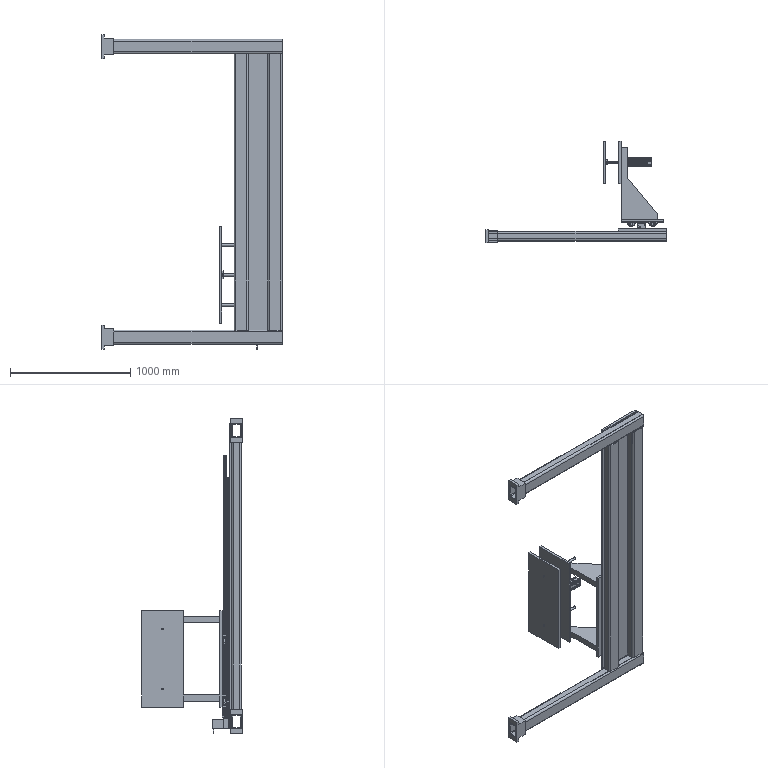Assembly | SolidWorks | mm | 26 component files | 26 solids | 1495 faces | box 1500 x 840 x 2621.5 mm | volume 76964541 mm3 | plane 802 | cylinder 635 | cone 42 | spline 16 | commonest cylinder face diameters 11 x160 7 x154 8 x48 5.5 x42 4.6 x24 4.26 x18 32 x16 16 x16
Bill of materials:
CQ2A50-200DCZ(0_0_0)1 | 1 |  | Long prismatic profile with a square-like cross-section. Each of the four corners has a rounded lobe with a round through-hole along the length. There are long grooves/slots on the faces and a small rectangular tab sticking out from one side at one end.
CQ2A50-200DCZ(0_0_0)2 | 1 |  | Headed pin: a long cylindrical shank with a thin, flat, round head at one end and a small step or chamfer at the other end.
HG_BLOCK_HGWHC_ANY | 4 |  | Block with a wide top flange and a narrower tapered lower body. A central open channel runs lengthwise through the underside. The flange has four through-holes and the side faces have curved pockets.
HG_RAIL0_R_ANY_1 | 2 |  | Very long, slender prismatic bar with a constant, complex cross-section. Concave semicircular notches are cut into the upper side edges, the lower part is chamfered, and there are two shallow notches in the bottom face.
LEFB32T-1800(0_0_0)1 | 1 |  | Long, slender L-shaped member: a straight bar with a short foot bent at one end. One view shows a broad rectangular face with rounded side edges, two small bosses and a small hole near one corner.
LEFB32T-1800(0_0_0)2 | 1 |  | Thin rectangular plate or cap with slightly tapered, rounded ends. Two longitudinal grooves run along its main face, and the edges are stepped.
ST60-02 | 2 |  | Straight rectangular hollow tube with rounded outer and inner corners and square-cut ends.
ST60-03 | 2 |  | Short rectangular hollow box section attached to a flat square plate at one end. The plate extends beyond the tube walls.
ST60-04 | 2 |  | Long rectangular hollow tube with rounded corners, uniform wall thickness and square-cut ends.
ST60-05 | 1 |  | Thin, flat, long rectangular strip of uniform thickness with no visible holes or cutouts.
ST60-06 | 1 |  | Thin, flat rectangular plate of uniform thickness with no visible holes, cutouts or edge features.
ST60-07 | 2 |  | Flat plate of uniform thickness shaped like a gusset: a narrow straight strip that widens along an angled edge into a broad, roughly trapezoidal end.
ST60-08 | 1 |  | Thin flat rectangular plate with three through holes in a line along the long centerline: a larger hole in the middle and a smaller hole near each end.
ST60-10 | 1 |  | Thin flat rectangular plate, similar in outline to a plain panel, with two very small holes on the long centerline, one near each end.
ST60-11 | 2 |  | Plain solid round rod or cylinder, long relative to its diameter, with flat ends.
ST60-12 | 1 |  | Thick rectangular block with a U-shaped slot open on one long side at mid-length and a round through hole on each side of the slot. A small step is visible near the slot opening.
ST60-13 | 1 |  | Hollow round tube with a short, larger-diameter flange at one end and a through bore along its axis, like a flanged sleeve or bushing.
Mates:
1. coincident | ST60-02-1 face at (-847.007, 19.454, 44) dir (-1, 0, 0) | ST60-03-1 face at (-847.007, 45.454, 100) dir (-1, 0, 0)
2. coincident | ST60-02-1 face at (652.993, -44.546, -44) dir (0, -1, 0) | ST60-03-1 face at (-847.007, -44.546, -60) dir (0, 1, 0)
3. coincident | ST60-02-1 face at (652.993, 19.454, 60) dir (0, 0, 1) | ST60-03-1 face at (-847.007, -44.546, 60) dir (0, 0, -1)
4. coincident | ST60-02-3 face at (652.993, 35.454, -2376) dir (0, 1, 0) | ST60-03-2 face at (-847.007, 35.454, -2480) dir (0, -1, 0)
5. coincident | ST60-02-3 face at (652.993, 19.454, -2360) dir (0, 0, 1) | ST60-03-2 face at (-847.007, -44.546, -2360) dir (0, 0, -1)
6. coincident | ST60-02-3 face at (-847.007, 19.454, -2376) dir (-1, 0, 0) | ST60-03-2 face at (-847.007, 45.454, -2320) dir (-1, 0, 0)
7. coincident | ST60-02-1 face at (652.993, -28.546, -60) dir (0, 0, -1) | ST60-04-1 face at (548.993, 19.454, -60) dir (0, 0, 1)
8. coincident | ST60-02-1 face at (652.993, -44.546, -44) dir (0, -1, 0) | ST60-04-1 face at (636.993, -44.546, -60) dir (0, -1, 0)
9. coincident | ST60-02-1 face at (652.993, 19.454, 44) dir (1, 0, 0) | ST60-04-1 face at (652.993, -28.546, -60) dir (1, 0, 0)
10. coincident | ST60-02-1 face at (652.993, -44.546, -44) dir (0, -1, 0) | ST60-02-3 face at (652.993, -44.546, -2464) dir (0, -1, 0)
11. coincident | ST60-02-1 face at (652.993, 19.454, 44) dir (1, 0, 0) | ST60-02-3 face at (652.993, 19.454, -2376) dir (1, 0, 0)
12. coincident | ST60-02-3 face at (652.993, 19.454, -2360) dir (0, 0, 1) | ST60-04-1 face at (548.993, 19.454, -2360) dir (0, 0, -1)
13. coincident | ST60-02-1 face at (652.993, -44.546, -44) dir (0, -1, 0) | ST60-04-2 face at (356.993, -44.546, -60) dir (0, -1, 0)
14. coincident | ST60-02-1 face at (652.993, -28.546, -60) dir (0, 0, -1) | ST60-04-2 face at (268.993, 19.454, -60) dir (0, 0, 1)
15. coincident | ST60-02-3 face at (652.993, -28.546, -2480) dir (0, 0, -1) | ST60-05-1 face at (252.993, 35.454, -2480) dir (0, 0, -1)
16. coincident | ST60-04-1 face at (652.993, -28.546, -60) dir (1, 0, 0) | ST60-05-1 face at (652.993, 35.454, -2480) dir (1, 0, 0)
17. coincident | ST60-02-3 face at (652.993, 35.454, -2376) dir (0, 1, 0) | ST60-05-1 face at (969.968, 35.454, -955.511) dir (0, -1, 0)
18. parallel | HG_RAIL0_R_ANY_1-1 face at (351.493, 101.454, -2378.228) dir (0, 1, 0) | HG_BLOCK_HGWHC_ANY-2 face at (357.193, 115.254, -2189.672) dir (0, 1, 0)
19. concentric | HG_RAIL0_R_ANY_1-1 face at (373.988, 100.949, -2346.4) dir (0, 0, 1) r 2.3 | HG_BLOCK_HGWHC_ANY-2 face at (373.988, 100.949, -2194.795) dir (0, 0, -1) r 2.3
20. coincident | HG_BLOCK_HGWHC_ANY-1 face at (380.493, 114.954, -1710.8) dir (0, 1, 0) | HG_BLOCK_HGWHC_ANY-2 face at (380.493, 114.954, -2210.8) dir (0, 1, 0)
21. coincident | HG_BLOCK_HGWHC_ANY-1 face at (397.993, 115.454, -1634.444) dir (1, 0, 0) | HG_BLOCK_HGWHC_ANY-2 face at (397.993, 115.454, -2134.444) dir (1, 0, 0)
22. distance | HG_BLOCK_HGWHC_ANY-2 face at (351.493, 79.454, -2301.4) dir (0, 0, -1) | HG_RAIL0_R_ANY_1-1 face at (351.999, 91.91, -2351.4) dir (0, 0, -1)
23. distance | HG_BLOCK_HGWHC_ANY-1 face at (351.493, 79.454, -1801.4) dir (0, 0, -1) | HG_BLOCK_HGWHC_ANY-2 face at (351.493, 79.454, -2301.4) dir (0, 0, -1)
24. distance | HG_RAIL0_R_ANY_1-1 face at (351.999, 91.91, -2351.4) dir (0, 0, -1) | LEFB32T-1800(0_0_0)-1/LEFB32T-1800(0_0_0)1-1 face at (478.951, 100.254, -2401.4) dir (0, 0, 1)
25. coincident | LEFB32T-1800(0_0_0)-1/LEFB32T-1800(0_0_0)2-1 face at (447.151, 115.454, -2390.4) dir (0, 1, 0) | ST60-06-1 face at (994.968, 115.454, -776.911) dir (0, -1, 0)
26. coincident | HG_BLOCK_HGWHC_ANY-2 face at (327.993, 115.454, -2134.444) dir (0, 1, 0) | ST60-06-1 face at (994.968, 115.454, -776.911) dir (0, -1, 0)
27. distance | HG_BLOCK_HGWHC_ANY-2 face at (327.993, 115.454, -2134.444) dir (-1, 0, 0) | ST60-06-1 face at (277.993, 115.454, -2301.4) dir (-1, 0, 0)
28. coincident | HG_BLOCK_HGWHC_ANY-1 face at (327.993, 115.454, -1634.444) dir (-1, 0, 0) | HG_BLOCK_HGWHC_ANY-2 face at (327.993, 115.454, -2134.444) dir (-1, 0, 0)
29. coincident | HG_BLOCK_HGWHC_ANY-3 face at (507.993, 115.454, -1634.444) dir (0, 1, 0) | HG_BLOCK_HGWHC_ANY-4 face at (507.993, 115.454, -2134.444) dir (0, 1, 0)
30. coincident | HG_BLOCK_HGWHC_ANY-3 face at (507.993, 115.454, -1634.444) dir (-1, 0, 0) | HG_BLOCK_HGWHC_ANY-4 face at (507.993, 115.454, -2134.444) dir (-1, 0, 0)
31. concentric | HG_RAIL0_R_ANY_1-2 face at (531.999, 100.949, -2346.4) dir (0, 0, 1) r 2.3 | HG_BLOCK_HGWHC_ANY-3 face at (531.999, 100.949, -1694.795) dir (0, 0, -1) r 2.3
32. parallel | HG_RAIL0_R_ANY_1-2 face at (531.493, 101.454, -2378.228) dir (0, 1, 0) | HG_BLOCK_HGWHC_ANY-3 face at (507.993, 115.454, -1634.444) dir (0, 1, 0)
33. coincident | ST60-06-1 face at (994.968, 115.454, -776.911) dir (0, -1, 0) | HG_BLOCK_HGWHC_ANY-4 face at (507.993, 115.454, -2134.444) dir (0, 1, 0)
34. coincident | HG_RAIL0_R_ANY_1-1 face at (373.988, 91.91, -211.4) dir (0, 0, 1) | HG_RAIL0_R_ANY_1-2 face at (553.988, 91.91, -211.4) dir (0, 0, 1)
35. coincident | HG_BLOCK_HGWHC_ANY-1 face at (374.493, 79.454, -1698.8) dir (0, 0, 1) | HG_BLOCK_HGWHC_ANY-3 face at (554.493, 79.454, -1698.8) dir (0, 0, 1)
36. coincident | HG_BLOCK_HGWHC_ANY-2 face at (351.493, 79.454, -2301.4) dir (0, 0, -1) | HG_BLOCK_HGWHC_ANY-4 face at (531.493, 79.454, -2301.4) dir (0, 0, -1)
37. distance | HG_BLOCK_HGWHC_ANY-4 face at (577.993, 115.454, -2134.444) dir (1, 0, 0) | ST60-06-1 face at (627.993, 115.454, -2301.4) dir (1, 0, 0)
38. coincident | ST60-05-1 face at (969.968, 55.454, -955.511) dir (0, 1, 0) | LEFB32T-1800(0_0_0)-1/LEFB32T-1800(0_0_0)1-1 face at (480.151, 55.454, -2393.4) dir (0, -1, 0)
39. coincident | ST60-06-1 face at (994.968, 135.454, -776.911) dir (0, 1, 0) | ST60-07-1 face at (577.993, 135.454, -2251.4) dir (0, -1, 0)
40. parallel | ST60-06-1 face at (627.993, 115.454, -2301.4) dir (1, 0, 0) | ST60-07-1 face at (277.993, 135.454, -2251.4) dir (-1, 0, 0)
41. coincident | ST60-06-1 face at (277.993, 115.454, -2301.4) dir (-1, 0, 0) | ST60-07-1 face at (277.993, 135.454, -2251.4) dir (-1, 0, 0)
42. distance | ST60-07-1 face at (277.993, 135.454, -2251.4) dir (0, 0, -1) | ST60-06-1 face at (277.993, 115.454, -2301.4) dir (0, 0, -1)
43. coincident | ST60-06-1 face at (994.968, 135.454, -776.911) dir (0, 1, 0) | ST60-07-2 face at (577.993, 135.454, -1601.4) dir (0, -1, 0)
44. distance | ST60-07-2 face at (277.993, 135.454, -1551.4) dir (0, 0, 1) | ST60-06-1 face at (277.993, 115.454, -1501.4) dir (0, 0, 1)
45. coincident | ST60-07-1 face at (327.993, 735.454, -2251.4) dir (1, 0, 0) | ST60-07-2 face at (327.993, 735.454, -1601.4) dir (1, 0, 0)
46. coincident | ST60-07-1 face at (277.993, 135.454, -2251.4) dir (-1, 0, 0) | ST60-08-1 face at (277.993, 68.479, -776.911) dir (1, 0, 0)
47. width | ST60-08-1 face at (257.993, 785.454, -2301.4) dir (0, 0, -1) | ST60-08-1 face at (257.993, 785.454, -1501.4) dir (0, 0, 1) | ST60-07-2 face at (277.993, 135.454, -1551.4) dir (0, 0, 1) | ST60-07-1 face at (277.993, 135.454, -2251.4) dir (0, 0, -1)
48. coincident | ST60-07-2 face at (277.993, 135.454, -1601.4) dir (-1, 0, 0) | ST60-08-1 face at (277.993, 68.479, -776.911) dir (1, 0, 0)
49. distance | ST60-06-1 face at (277.993, 115.454, -2301.4) dir (0, 0, -1) | LEFB32T-1800(0_0_0)-1/LEFB32T-1800(0_0_0)1-1 face at (478.951, 100.254, -2401.4) dir (0, 0, 1)
50. distance | ST60-07-1 face at (277.993, 735.454, -2251.4) dir (0, 1, 0) | ST60-08-1 face at (257.993, 785.454, -2301.4) dir (0, 1, 0)
51. width | ST60-06-1 face at (627.993, 115.454, -2301.4) dir (1, 0, 0) | ST60-06-1 face at (277.993, 115.454, -2301.4) dir (-1, 0, 0) | ST60-05-1 face at (252.993, 35.454, -2480) dir (-1, 0, 0) | ST60-05-1 face at (652.993, 35.454, -2480) dir (1, 0, 0)
52. coincident | ST60-05-1 face at (252.993, 35.454, -2480) dir (0, 0, -1) | LEFB32T-1800(0_0_0)-1/LEFB32T-1800(0_0_0)1-1 face at (482.051, 55.954, -2480) dir (0, 0, -1)
53. coincident | ST60-04-2 face at (252.993, 19.454, -60) dir (-1, 0, 0) | ST60-05-1 face at (252.993, 35.454, -2480) dir (-1, 0, 0)
54. width | ST60-10-1 face at (131.993, 785.454, -2301.4) dir (0, 1, 0) | ST60-10-1 face at (131.993, 435.454, -2301.4) dir (0, -1, 0) | ST60-08-1 face at (257.993, 435.454, -2301.4) dir (0, -1, 0) | ST60-08-1 face at (257.993, 785.454, -2301.4) dir (0, 1, 0)
55. width | ST60-08-1 face at (257.993, 785.454, -2301.4) dir (0, 0, -1) | ST60-08-1 face at (257.993, 785.454, -1501.4) dir (0, 0, 1) | ST60-10-1 face at (131.993, 785.454, -1501.4) dir (0, 0, 1) | ST60-10-1 face at (131.993, 785.454, -2301.4) dir (0, 0, -1)
56. coincident | ST60-08-1 face at (277.993, 68.479, -776.911) dir (1, 0, 0) | CQ2A50-200DCZ(0_0_0)-1/CQ2A50-200DCZ(0_0_0)1-1 face at (277.993, 610.454, -1901.4) dir (-1, 0, 0)
57. concentric | ST60-08-1 face at (277.993, 610.454, -1651.4) dir (-1, 0, 0) r 10 | ST60-11-1 face at (151.993, 610.454, -1651.4) dir (1, 0, 0) r 10
58. coincident | ST60-08-1 edge at (277.993, 610.454, -2151.4) dir (-1, 0, 0) r 10 | ST60-11-2 face at (151.993, 610.454, -2151.4) dir (1, 0, 0) r 10
59. concentric | ST60-08-1 edge at (277.993, 610.454, -1901.4) dir (-1, 0, 0) r 17.5 | CQ2A50-200DCZ(0_0_0)-1/CQ2A50-200DCZ(0_0_0)1-1 edge at (533.493, 610.454, -1901.4) dir (-1, 0, 0) r 26
60. parallel | ST60-08-1 face at (257.993, 785.454, -2301.4) dir (0, 1, 0) | CQ2A50-200DCZ(0_0_0)-1/CQ2A50-200DCZ(0_0_0)1-1 face at (277.993, 649.454, -1891.9) dir (0, 1, 0)
61. coincident | ST60-10-1 face at (151.993, 68.479, -776.911) dir (1, 0, 0) | ST60-11-2 face at (151.993, 610.454, -2151.4) dir (-1, 0, 0)
62. coincident | ST60-10-1 face at (151.993, 68.479, -776.911) dir (1, 0, 0) | ST60-11-1 face at (151.993, 610.454, -1651.4) dir (-1, 0, 0)
63. concentric | ST60-13-1 face at (159.993, 610.454, -1901.4) dir (1, 0, 0) r 10 | ST60-12-1 edge at (165.193, 610.454, -1901.4) dir (1, 0, 0) r 10.2
64. coincident | ST60-13-1 face at (151.993, 610.454, -1901.4) dir (-1, 0, 0) | ST60-12-1 face at (151.993, 587.454, -1914.4) dir (-1, 0, 0)
65. concentric | ST60-08-1 face at (277.993, 610.454, -1901.4) dir (-1, 0, 0) r 17.5 | ST60-13-1 face at (151.993, 610.454, -1901.4) dir (1, 0, 0) r 12.5
66. coincident | ST60-10-1 face at (151.993, 68.479, -776.911) dir (1, 0, 0) | ST60-12-1 face at (151.993, 587.454, -1868.4) dir (-1, 0, 0)
67. parallel | ST60-10-1 face at (131.993, 785.454, -2301.4) dir (0, 1, 0) | ST60-12-1 face at (158.075, 633.454, -1900.01) dir (0, 1, 0)
68. coincident | CQ2A50-200DCZ(0_0_0)-1/CQ2A50-200DCZ(0_0_0)2-1 face at (259.993, 617.954, -1901.4) dir (-1, 0, 0) | ST60-13-1 face at (259.993, 610.454, -1901.4) dir (1, 0, 0)